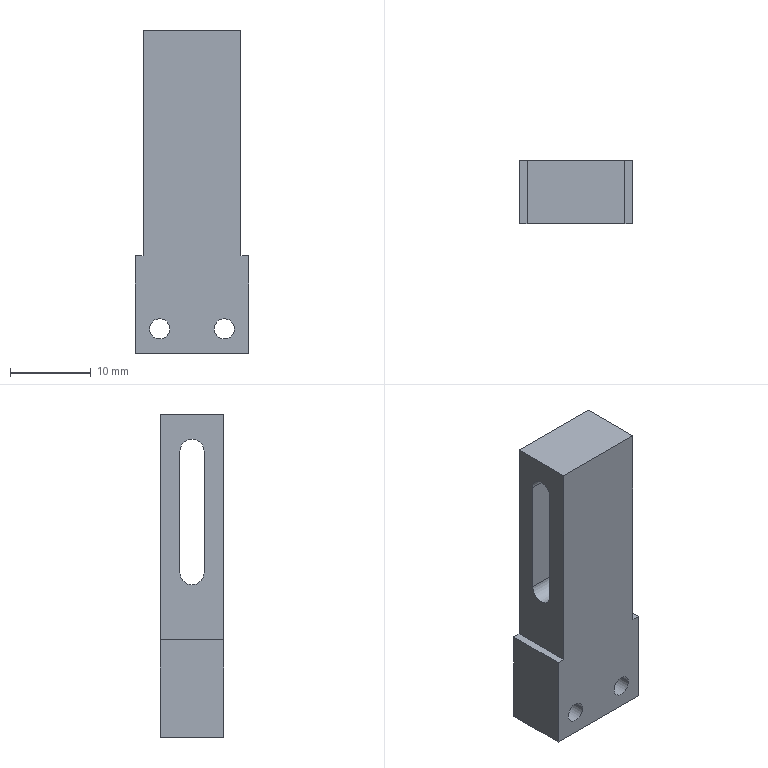Component | SolidWorks | ChainPartPhotoelectricSwitchBracket-1 | 1 solid | 19 faces | box 14 x 7.8 x 39.8 mm | volume 3228 mm3 | plane 12 | cylinder 7 | commonest cylinder face diameters 2.5 x4 3 x3
build123d program:
from build123d import *

# Parameters (mm, degrees)
SKETCH1_W           = 39.8
SKETCH1_H           = 7.8
BOSS_EXTRUDE1_DEPTH = 7
SKETCH2_W           = 27.8
SKETCH2_H           = 0.95
CUT_EXTRUDE1_DEPTH  = 23.491
M3_TAPPED_HOLE1_D   = 2.5
CUT_EXTRUDE2_DEPTH  = 25.115


with BuildPart() as part:
    # Sketch1 → Boss-Extrude1 (new, symmetric)
    with BuildSketch(Plane.XY):
        Rectangle(SKETCH1_W, SKETCH1_H)
    extrude(amount=BOSS_EXTRUDE1_DEPTH, both=True)

    # Sketch2 → Cut-Extrude1 (cut, through all)
    with BuildSketch(Plane(origin=(0, 3.9, 0), x_dir=(1, 0, 0), z_dir=(0, 1, 0))):
        with Locations((6, 6.525)):
            Rectangle(SKETCH2_W, SKETCH2_H)
        with Locations((6, -6.525)):
            Rectangle(SKETCH2_W, SKETCH2_H)
    extrude(amount=-CUT_EXTRUDE1_DEPTH, mode=Mode.SUBTRACT)

    # M3 Tapped Hole1 (through all)
    with Locations(Plane(origin=(0, 3.9, 0), x_dir=(-1, 0, 0), z_dir=(0, 1, 0))):
        with Locations((16.9, -4), (16.9, 4)):
            Hole(M3_TAPPED_HOLE1_D / 2)

    # Sketch5 → Cut-Extrude2 (cut, through all)
    with BuildSketch(Plane.XY.offset(6.05)):
        with BuildLine():
            Line((0.4, 1.5), (15.4, 1.5))
            ThreePointArc((15.4, 1.5), (16.9, 0), (15.4, -1.5))
            Line((15.4, -1.5), (0.4, -1.5))
            ThreePointArc((0.4, -1.5), (-1.1, 0), (0.4, 1.5))
        make_face()
    extrude(amount=-CUT_EXTRUDE2_DEPTH, mode=Mode.SUBTRACT)


solid = part.part

# Placed as in the assembly
solid = solid.moved(Location((141.687, -33.063, -287.454), (0, -90, 0)))